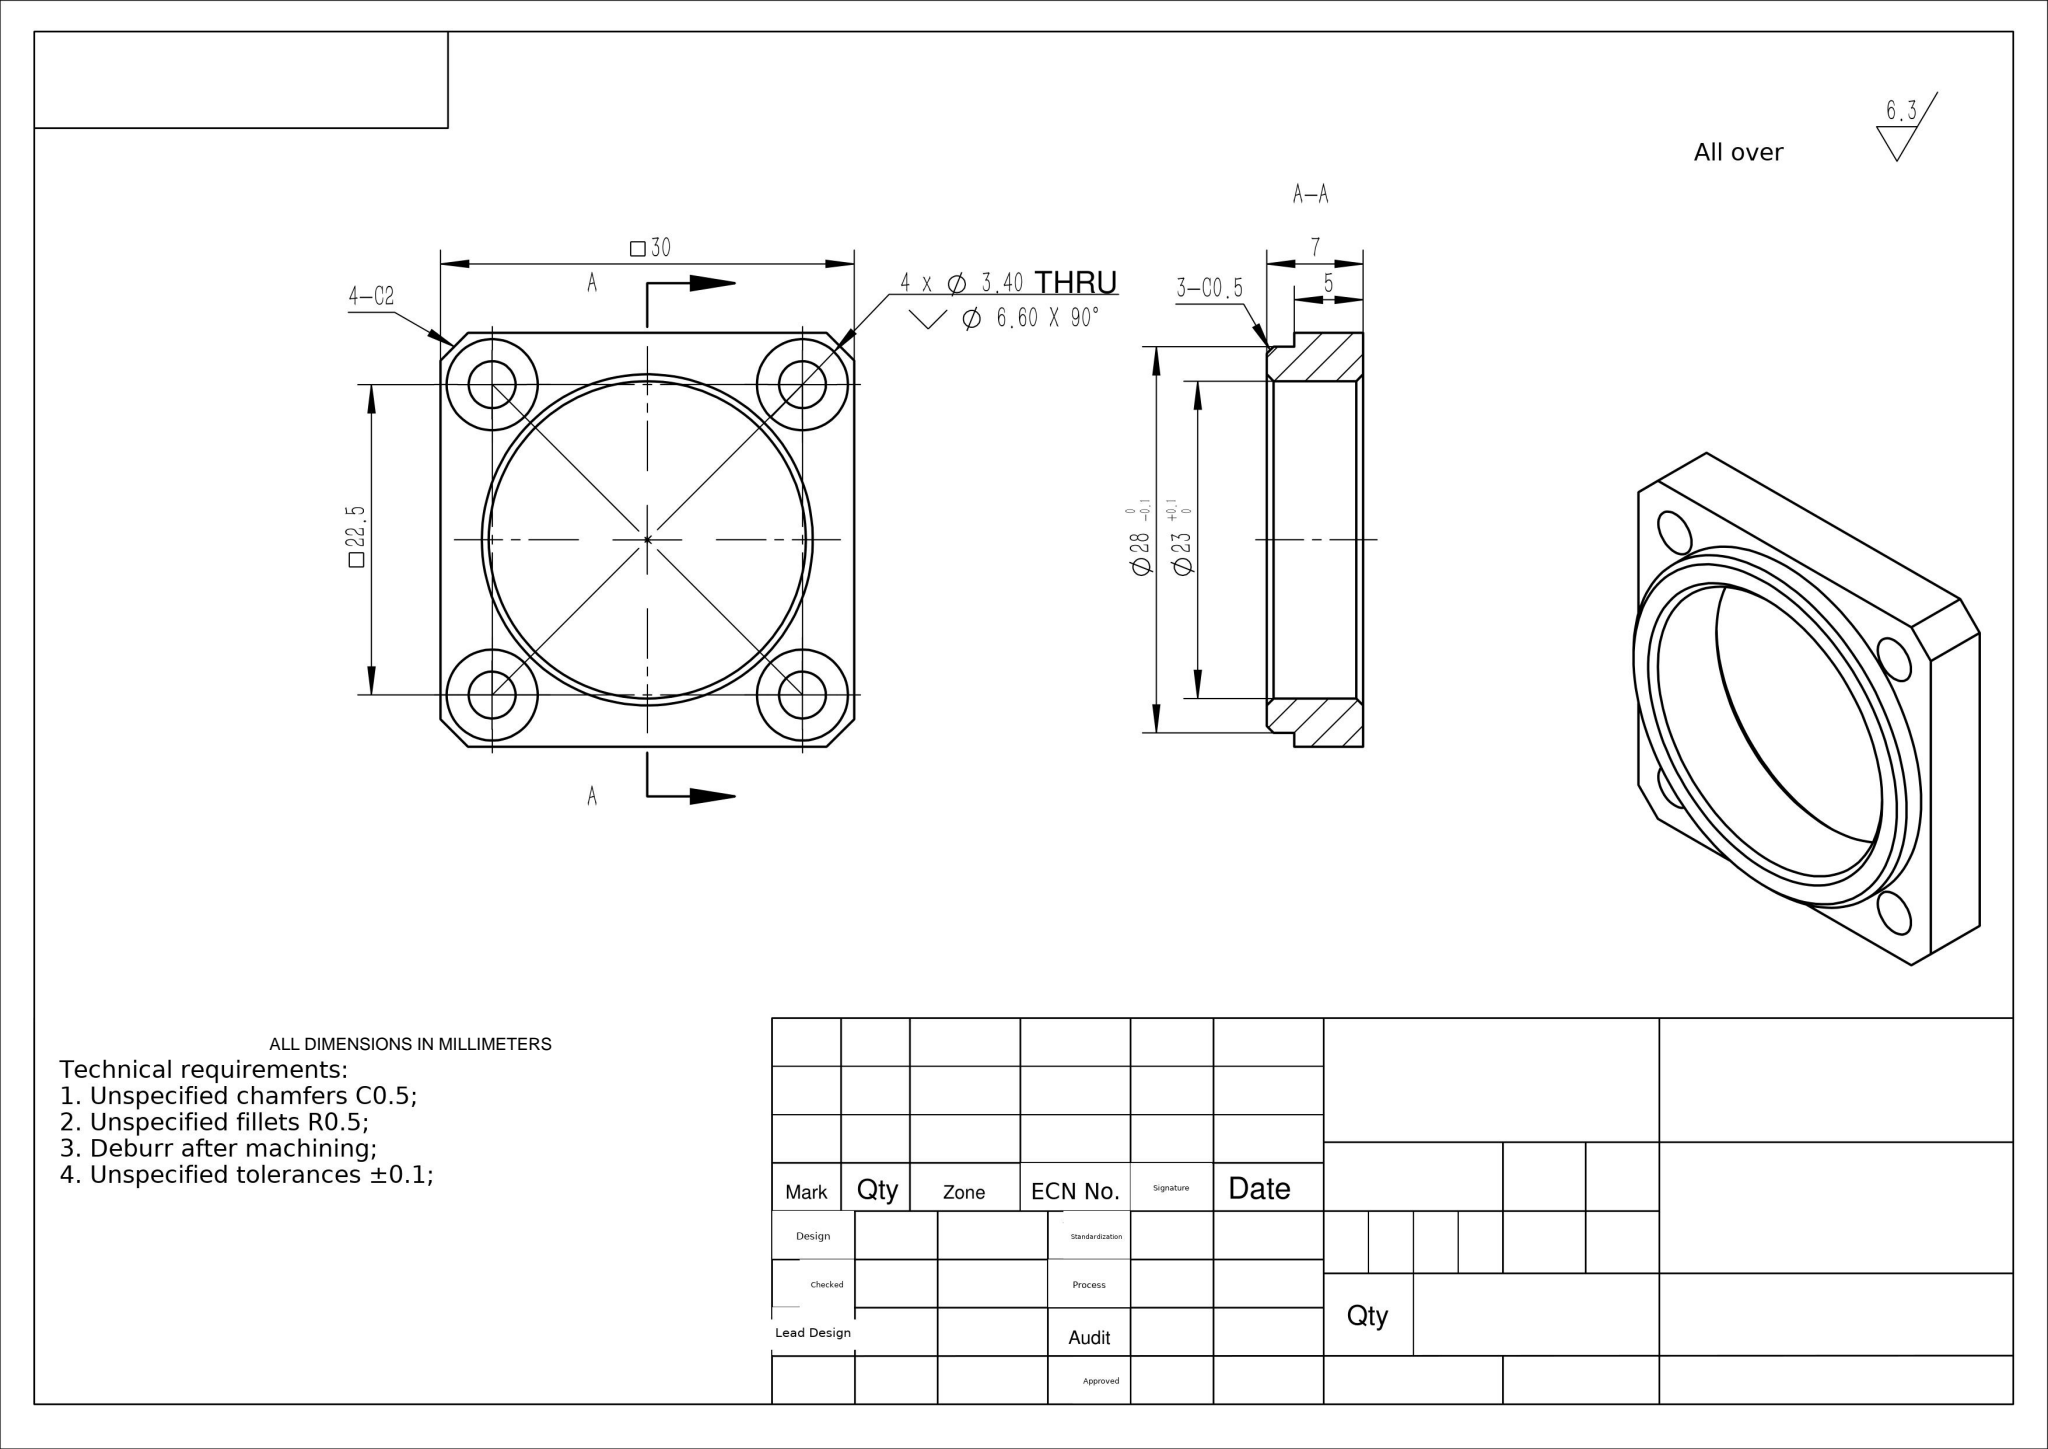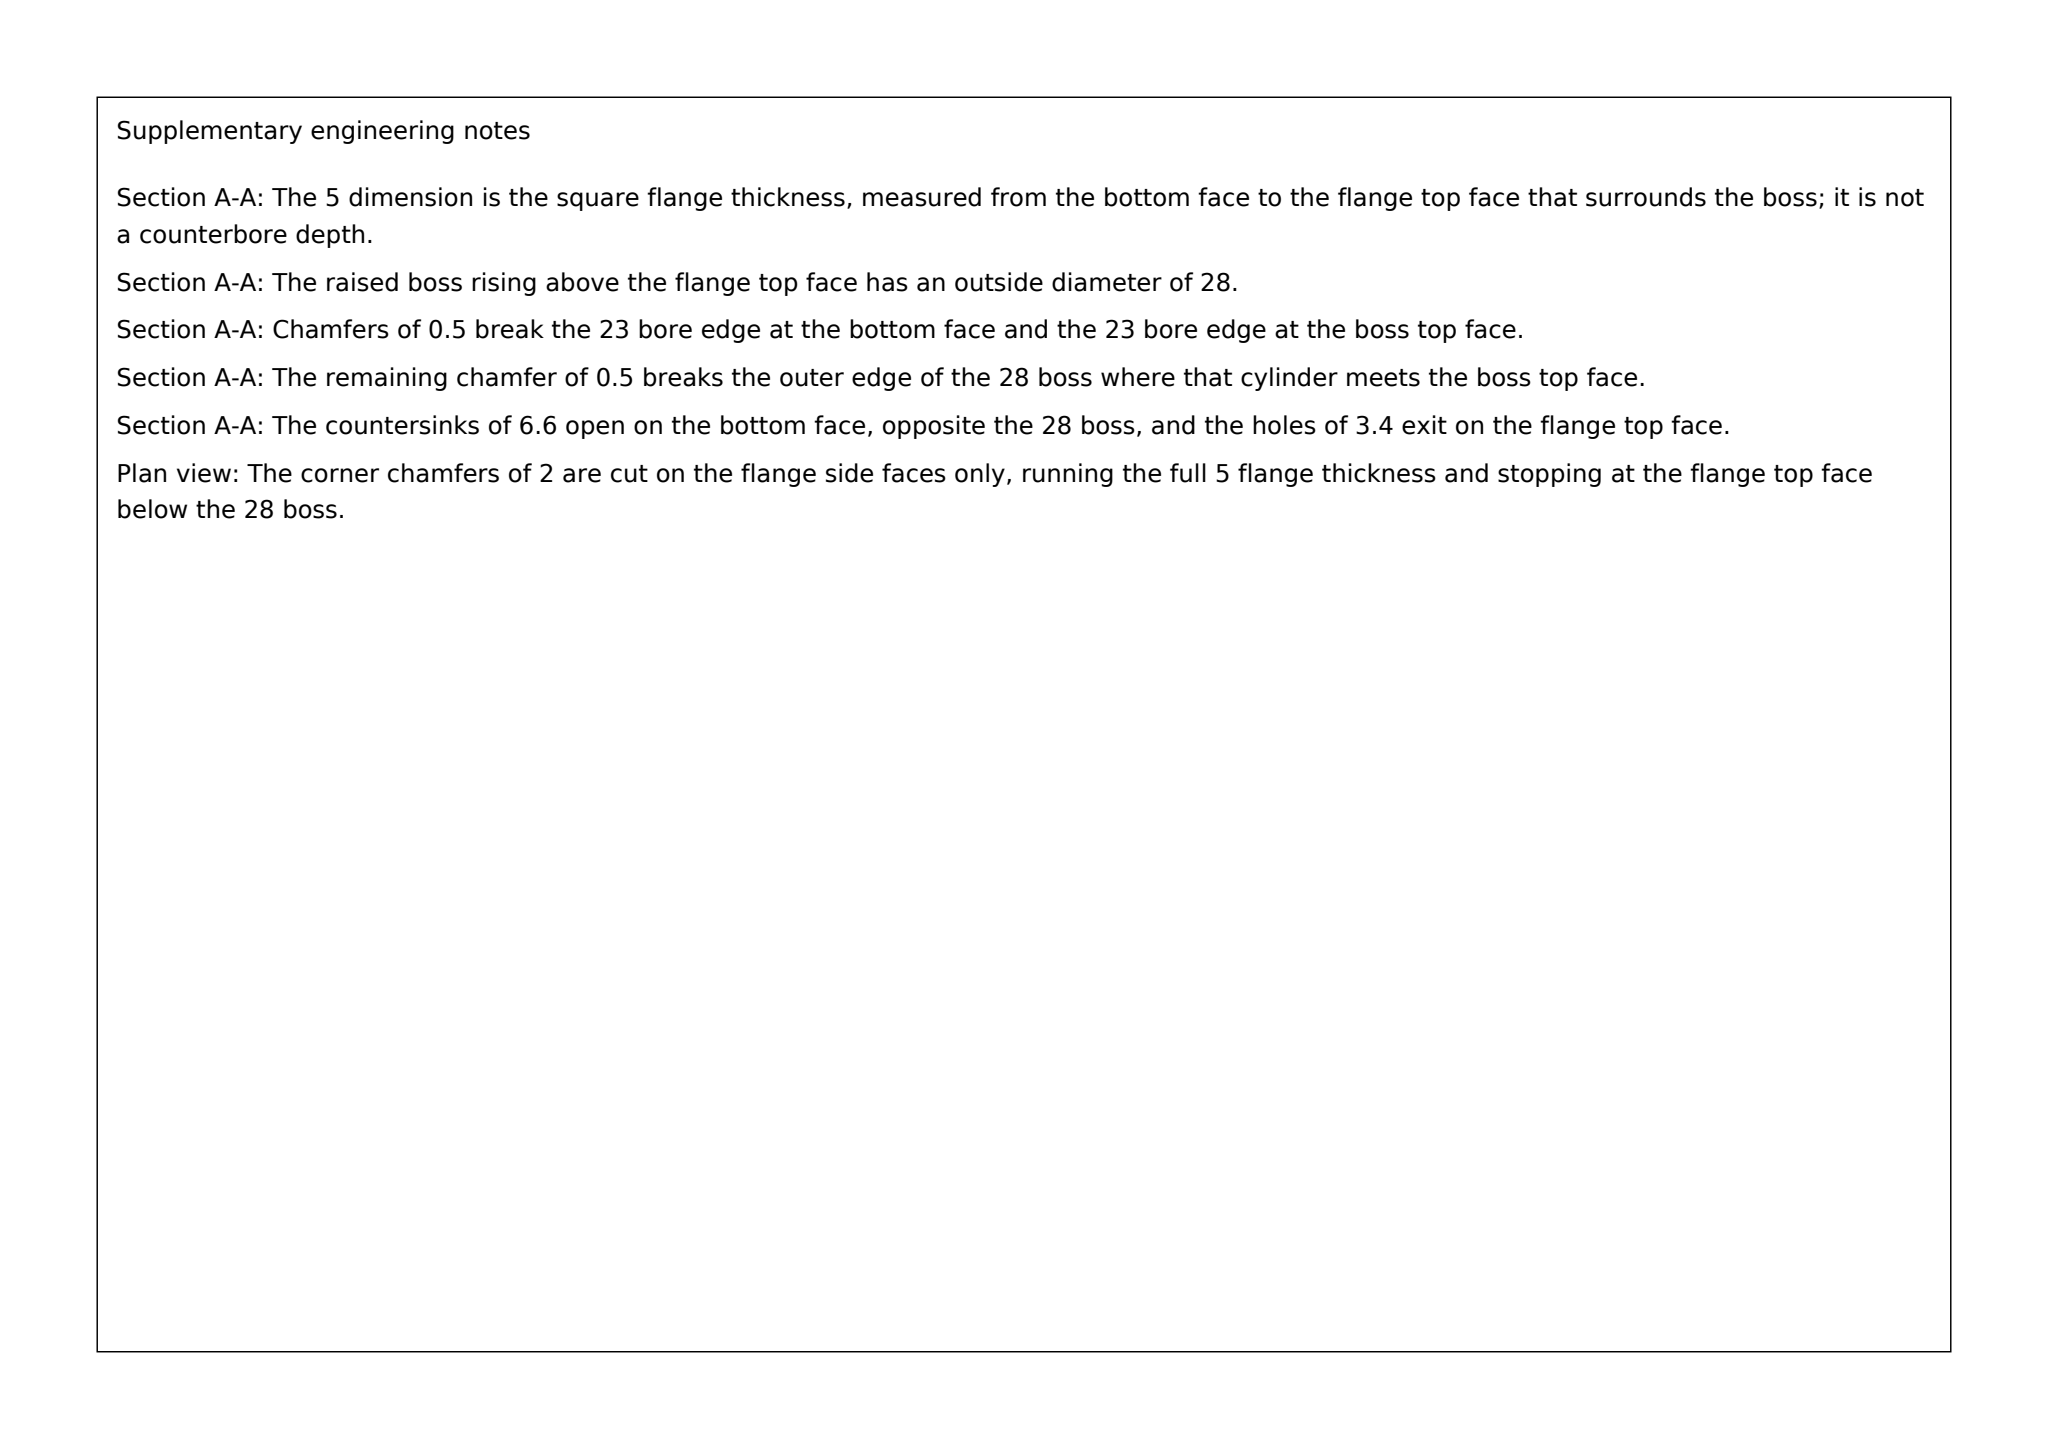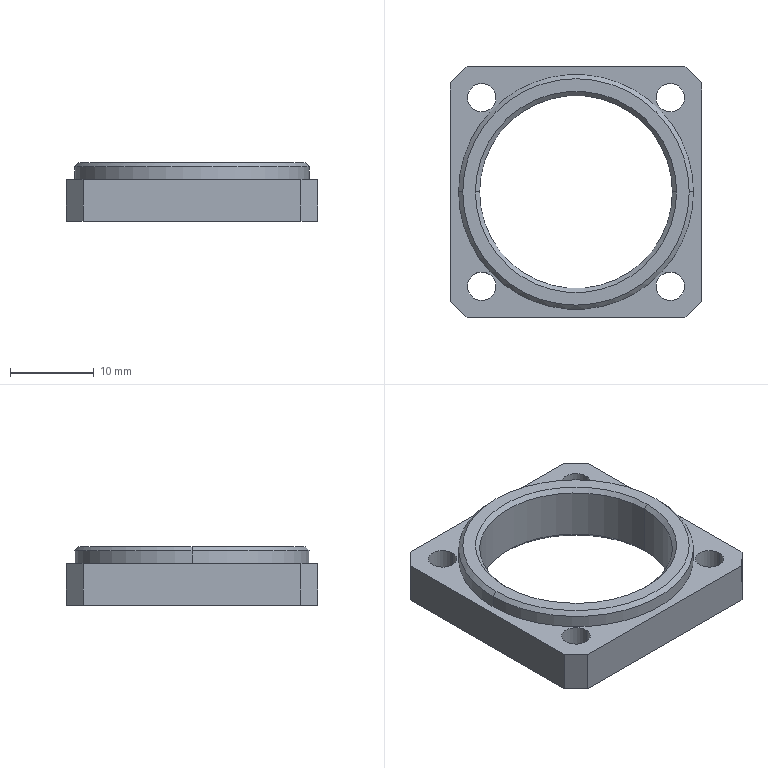Part | SolidWorks | mm | 1 solid | 37 faces | box 30 x 30 x 7 mm | volume 2501 mm3 | cone 14 | cylinder 12 | plane 11 | commonest cylinder face diameters 3.4 x8 28 x2 23 x2
build123d program:
from build123d import *

# Parameters (mm, degrees)
SKETCH1_W                                         = 30
SKETCH1_H                                         = 30
SKETCH1_R                                         = 11.5
BOSS_EXTRUDE1_DEPTH                               = 5
SKETCH3_R                                         = 14
SKETCH3_R_2                                       = 11.5
BOSS_EXTRUDE2_DEPTH                               = 2
HOLE_SIZE_ACCORDING_TO_PHILLIPS_RAISE_D           = 3.4
HOLE_SIZE_ACCORDING_TO_PHILLIPS_RAISE_CSINK_D     = 6.6
HOLE_SIZE_ACCORDING_TO_PHILLIPS_RAISE_CSINK_ANGLE = 90
CHAMFER1_SIZE                                     = 2
CHAMFER2_SIZE                                     = 0.5


with BuildPart() as part:
    # Sketch1 → Boss-Extrude1 (new body)
    with BuildSketch(Plane.XY):
        Rectangle(SKETCH1_W, SKETCH1_H)
        Circle(SKETCH1_R, mode=Mode.SUBTRACT)
    extrude(amount=BOSS_EXTRUDE1_DEPTH)

    # Sketch3 → Boss-Extrude2 (add)
    with BuildSketch(Plane.XY.offset(5)):
        Circle(SKETCH3_R)
        Circle(SKETCH3_R_2, mode=Mode.SUBTRACT)
    extrude(amount=BOSS_EXTRUDE2_DEPTH)

    # Hole Size _ according to Phillips_ Raise (through all)
    with Locations(Plane(origin=(0, 0, 0), x_dir=(-1, 0, 0), z_dir=(0, 0, -1))):
        with Locations((-11.25, 11.25), (11.25, 11.25), (11.25, -11.25), (-11.25, -11.25)):
            CounterSinkHole(HOLE_SIZE_ACCORDING_TO_PHILLIPS_RAISE_D / 2, HOLE_SIZE_ACCORDING_TO_PHILLIPS_RAISE_CSINK_D / 2, counter_sink_angle=HOLE_SIZE_ACCORDING_TO_PHILLIPS_RAISE_CSINK_ANGLE)

    # Chamfer1
    chamfer1_edges = [part.edges().sort_by_distance(p)[0] for p in [
        (-15, 15, 2.5),
        (15, 15, 2.5),
        (15, -15, 2.5),
        (-15, -15, 2.5),
    ]]
    chamfer(chamfer1_edges, length=CHAMFER1_SIZE)

    # Chamfer2
    chamfer2_edges = [part.edges().sort_by_distance(p)[0] for p in [
        (-11.5, 0, 0),
        (-14, 0, 7),
        (-11.5, 0, 7),
    ]]
    chamfer(chamfer2_edges, length=CHAMFER2_SIZE)


solid = part.part